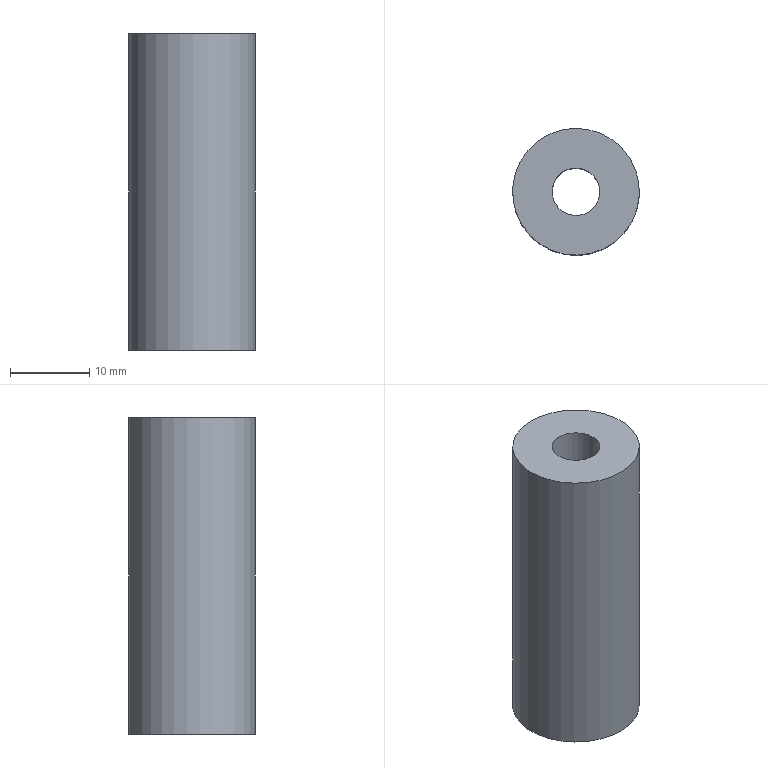Component | NX | 2 | 1 solid | 4 faces | box 16 x 16 x 40 mm | volume 6912 mm3 | cylinder 2 | plane 2 | commonest cylinder face diameters 16 x1 6 x1
STEP:
#1=CARTESIAN_POINT('',(0.,0.,0.));
#2=DIRECTION('',(0.,0.,1.));
#3=DIRECTION('',(1.,0.,0.));
#4=AXIS2_PLACEMENT_3D('',#1,#2,#3);
#5=CARTESIAN_POINT('',(376.69,35.694,0.));
#6=VERTEX_POINT('',#5);
#7=CARTESIAN_POINT('',(369.673,39.537,0.));
#8=DIRECTION('',(0.,0.,-1.));
#9=DIRECTION('',(0.8771,-0.4803,0.));
#10=AXIS2_PLACEMENT_3D('',#7,#8,#9);
#11=CIRCLE('',#10,8.);
#12=CARTESIAN_POINT('',(369.673,39.537,0.));
#13=DIRECTION('',(0.,0.,1.));
#14=DIRECTION('',(-0.8771,0.4803,0.));
#15=AXIS2_PLACEMENT_3D('',#12,#13,#14);
#16=CYLINDRICAL_SURFACE('',#15,8.);
#17=CARTESIAN_POINT('',(9.425,0.));
#18=DIRECTION('',(-1.,0.));
#19=VECTOR('',#18,1.);
#20=LINE('',#17,#19);
#21=(GEOMETRIC_REPRESENTATION_CONTEXT(2)PARAMETRIC_REPRESENTATION_CONTEXT()REPRESENTATION_CONTEXT('',''));
#22=DEFINITIONAL_REPRESENTATION('',(#20),#21);
#23=PCURVE('',#16,#22);
#24=CARTESIAN_POINT('',(369.673,39.537,0.));
#25=DIRECTION('',(0.,0.,-1.));
#26=DIRECTION('',(0.8771,-0.4803,0.));
#27=AXIS2_PLACEMENT_3D('',#24,#25,#26);
#28=PLANE('',#27);
#29=CARTESIAN_POINT('',(0.,0.));
#30=DIRECTION('',(1.,0.));
#31=AXIS2_PLACEMENT_2D('',#29,#30);
#32=CIRCLE('',#31,8.);
#33=(GEOMETRIC_REPRESENTATION_CONTEXT(2)PARAMETRIC_REPRESENTATION_CONTEXT()REPRESENTATION_CONTEXT('',''));
#34=DEFINITIONAL_REPRESENTATION('',(#32),#33);
#35=PCURVE('',#28,#34);
#36=SURFACE_CURVE('',#11,(#23,#35),.PCURVE_S1.);
#37=EDGE_CURVE('',#6,#6,#36,.T.);
#38=ORIENTED_EDGE('',*,*,#37,.F.);
#39=CARTESIAN_POINT('',(376.69,35.694,40.));
#40=VERTEX_POINT('',#39);
#41=CARTESIAN_POINT('',(376.69,35.694,0.));
#42=CARTESIAN_POINT('',(376.69,35.694,40.));
#43=B_SPLINE_CURVE_WITH_KNOTS('',1,(#41,#42),.UNSPECIFIED.,.F.,.F.,(2,2),(0.,40.),.PIECEWISE_BEZIER_KNOTS.);
#44=CARTESIAN_POINT('',(9.425,0.));
#45=DIRECTION('',(0.,1.));
#46=VECTOR('',#45,1.);
#47=LINE('',#44,#46);
#48=(GEOMETRIC_REPRESENTATION_CONTEXT(2)PARAMETRIC_REPRESENTATION_CONTEXT()REPRESENTATION_CONTEXT('',''));
#49=DEFINITIONAL_REPRESENTATION('',(#47),#48);
#50=PCURVE('',#16,#49);
#51=CARTESIAN_POINT('',(3.142,0.));
#52=DIRECTION('',(0.,1.));
#53=VECTOR('',#52,1.);
#54=LINE('',#51,#53);
#55=(GEOMETRIC_REPRESENTATION_CONTEXT(2)PARAMETRIC_REPRESENTATION_CONTEXT()REPRESENTATION_CONTEXT('',''));
#56=DEFINITIONAL_REPRESENTATION('',(#54),#55);
#57=PCURVE('',#16,#56);
#58=SEAM_CURVE('',#43,(#50,#57),.PCURVE_S1.);
#59=EDGE_CURVE('',#6,#40,#58,.T.);
#60=ORIENTED_EDGE('',*,*,#59,.T.);
#61=CARTESIAN_POINT('',(369.673,39.537,40.));
#62=DIRECTION('',(0.,0.,-1.));
#63=DIRECTION('',(0.8771,-0.4803,0.));
#64=AXIS2_PLACEMENT_3D('',#61,#62,#63);
#65=CIRCLE('',#64,8.);
#66=CARTESIAN_POINT('',(9.425,40.));
#67=DIRECTION('',(-1.,0.));
#68=VECTOR('',#67,1.);
#69=LINE('',#66,#68);
#70=(GEOMETRIC_REPRESENTATION_CONTEXT(2)PARAMETRIC_REPRESENTATION_CONTEXT()REPRESENTATION_CONTEXT('',''));
#71=DEFINITIONAL_REPRESENTATION('',(#69),#70);
#72=PCURVE('',#16,#71);
#73=CARTESIAN_POINT('',(369.673,39.537,40.));
#74=DIRECTION('',(0.,0.,-1.));
#75=DIRECTION('',(0.8771,-0.4803,0.));
#76=AXIS2_PLACEMENT_3D('',#73,#74,#75);
#77=PLANE('',#76);
#78=CARTESIAN_POINT('',(0.,0.));
#79=DIRECTION('',(1.,0.));
#80=AXIS2_PLACEMENT_2D('',#78,#79);
#81=CIRCLE('',#80,8.);
#82=(GEOMETRIC_REPRESENTATION_CONTEXT(2)PARAMETRIC_REPRESENTATION_CONTEXT()REPRESENTATION_CONTEXT('',''));
#83=DEFINITIONAL_REPRESENTATION('',(#81),#82);
#84=PCURVE('',#77,#83);
#85=SURFACE_CURVE('',#65,(#72,#84),.PCURVE_S1.);
#86=EDGE_CURVE('',#40,#40,#85,.T.);
#87=ORIENTED_EDGE('',*,*,#86,.T.);
#88=ORIENTED_EDGE('',*,*,#59,.F.);
#89=EDGE_LOOP('',(#38,#60,#87,#88));
#90=FACE_BOUND('',#89,.T.);
#91=ADVANCED_FACE('',(#90),#16,.T.);
#92=CARTESIAN_POINT('',(372.304,38.096,0.));
#93=VERTEX_POINT('',#92);
#94=CARTESIAN_POINT('',(369.673,39.537,0.));
#95=DIRECTION('',(0.,0.,-1.));
#96=DIRECTION('',(0.8771,-0.4803,0.));
#97=AXIS2_PLACEMENT_3D('',#94,#95,#96);
#98=CIRCLE('',#97,3.);
#99=CARTESIAN_POINT('',(369.673,39.537,0.));
#100=DIRECTION('',(0.,0.,1.));
#101=DIRECTION('',(-0.8771,0.4803,0.));
#102=AXIS2_PLACEMENT_3D('',#99,#100,#101);
#103=CYLINDRICAL_SURFACE('',#102,3.);
#104=CARTESIAN_POINT('',(9.425,0.));
#105=DIRECTION('',(-1.,0.));
#106=VECTOR('',#105,1.);
#107=LINE('',#104,#106);
#108=(GEOMETRIC_REPRESENTATION_CONTEXT(2)PARAMETRIC_REPRESENTATION_CONTEXT()REPRESENTATION_CONTEXT('',''));
#109=DEFINITIONAL_REPRESENTATION('',(#107),#108);
#110=PCURVE('',#103,#109);
#111=CARTESIAN_POINT('',(0.,0.));
#112=DIRECTION('',(1.,0.));
#113=AXIS2_PLACEMENT_2D('',#111,#112);
#114=CIRCLE('',#113,3.);
#115=(GEOMETRIC_REPRESENTATION_CONTEXT(2)PARAMETRIC_REPRESENTATION_CONTEXT()REPRESENTATION_CONTEXT('',''));
#116=DEFINITIONAL_REPRESENTATION('',(#114),#115);
#117=PCURVE('',#28,#116);
#118=SURFACE_CURVE('',#98,(#110,#117),.PCURVE_S1.);
#119=EDGE_CURVE('',#93,#93,#118,.T.);
#120=ORIENTED_EDGE('',*,*,#119,.F.);
#121=CARTESIAN_POINT('',(372.304,38.096,40.));
#122=VERTEX_POINT('',#121);
#123=CARTESIAN_POINT('',(372.304,38.096,0.));
#124=CARTESIAN_POINT('',(372.304,38.096,40.));
#125=B_SPLINE_CURVE_WITH_KNOTS('',1,(#123,#124),.UNSPECIFIED.,.F.,.F.,(2,2),(0.,40.),.PIECEWISE_BEZIER_KNOTS.);
#126=CARTESIAN_POINT('',(9.425,0.));
#127=DIRECTION('',(0.,1.));
#128=VECTOR('',#127,1.);
#129=LINE('',#126,#128);
#130=(GEOMETRIC_REPRESENTATION_CONTEXT(2)PARAMETRIC_REPRESENTATION_CONTEXT()REPRESENTATION_CONTEXT('',''));
#131=DEFINITIONAL_REPRESENTATION('',(#129),#130);
#132=PCURVE('',#103,#131);
#133=CARTESIAN_POINT('',(3.142,0.));
#134=DIRECTION('',(0.,1.));
#135=VECTOR('',#134,1.);
#136=LINE('',#133,#135);
#137=(GEOMETRIC_REPRESENTATION_CONTEXT(2)PARAMETRIC_REPRESENTATION_CONTEXT()REPRESENTATION_CONTEXT('',''));
#138=DEFINITIONAL_REPRESENTATION('',(#136),#137);
#139=PCURVE('',#103,#138);
#140=SEAM_CURVE('',#125,(#132,#139),.PCURVE_S1.);
#141=EDGE_CURVE('',#93,#122,#140,.T.);
#142=ORIENTED_EDGE('',*,*,#141,.T.);
#143=CARTESIAN_POINT('',(369.673,39.537,40.));
#144=DIRECTION('',(0.,0.,-1.));
#145=DIRECTION('',(0.8771,-0.4803,0.));
#146=AXIS2_PLACEMENT_3D('',#143,#144,#145);
#147=CIRCLE('',#146,3.);
#148=CARTESIAN_POINT('',(9.425,40.));
#149=DIRECTION('',(-1.,0.));
#150=VECTOR('',#149,1.);
#151=LINE('',#148,#150);
#152=(GEOMETRIC_REPRESENTATION_CONTEXT(2)PARAMETRIC_REPRESENTATION_CONTEXT()REPRESENTATION_CONTEXT('',''));
#153=DEFINITIONAL_REPRESENTATION('',(#151),#152);
#154=PCURVE('',#103,#153);
#155=CARTESIAN_POINT('',(0.,0.));
#156=DIRECTION('',(1.,0.));
#157=AXIS2_PLACEMENT_2D('',#155,#156);
#158=CIRCLE('',#157,3.);
#159=(GEOMETRIC_REPRESENTATION_CONTEXT(2)PARAMETRIC_REPRESENTATION_CONTEXT()REPRESENTATION_CONTEXT('',''));
#160=DEFINITIONAL_REPRESENTATION('',(#158),#159);
#161=PCURVE('',#77,#160);
#162=SURFACE_CURVE('',#147,(#154,#161),.PCURVE_S1.);
#163=EDGE_CURVE('',#122,#122,#162,.T.);
#164=ORIENTED_EDGE('',*,*,#163,.T.);
#165=ORIENTED_EDGE('',*,*,#141,.F.);
#166=EDGE_LOOP('',(#120,#142,#164,#165));
#167=FACE_BOUND('',#166,.F.);
#168=ADVANCED_FACE('',(#167),#103,.F.);
#169=ORIENTED_EDGE('',*,*,#37,.T.);
#170=EDGE_LOOP('',(#169));
#171=FACE_BOUND('',#170,.T.);
#172=ORIENTED_EDGE('',*,*,#119,.F.);
#173=EDGE_LOOP('',(#172));
#174=FACE_BOUND('',#173,.T.);
#175=ADVANCED_FACE('',(#171,#174),#28,.T.);
#176=ORIENTED_EDGE('',*,*,#86,.F.);
#177=EDGE_LOOP('',(#176));
#178=FACE_BOUND('',#177,.T.);
#179=ORIENTED_EDGE('',*,*,#163,.T.);
#180=EDGE_LOOP('',(#179));
#181=FACE_BOUND('',#180,.T.);
#182=ADVANCED_FACE('',(#178,#181),#77,.F.);
#183=CLOSED_SHELL('',(#91,#168,#175,#182));
#184=MANIFOLD_SOLID_BREP('',#183);
#185=(LENGTH_UNIT()NAMED_UNIT(*)SI_UNIT(.MILLI.,.METRE.));
#186=UNCERTAINTY_MEASURE_WITH_UNIT(LENGTH_MEASURE(0.00001),#185,'','');
#187=(NAMED_UNIT(*)PLANE_ANGLE_UNIT()SI_UNIT($,.RADIAN.));
#188=(NAMED_UNIT(*)SI_UNIT($,.STERADIAN.)SOLID_ANGLE_UNIT());
#189=(GEOMETRIC_REPRESENTATION_CONTEXT(3)GLOBAL_UNCERTAINTY_ASSIGNED_CONTEXT((#186))GLOBAL_UNIT_ASSIGNED_CONTEXT((#185,#187,#188))REPRESENTATION_CONTEXT('',''));
#190=ADVANCED_BREP_SHAPE_REPRESENTATION('',(#4,#184),#189);